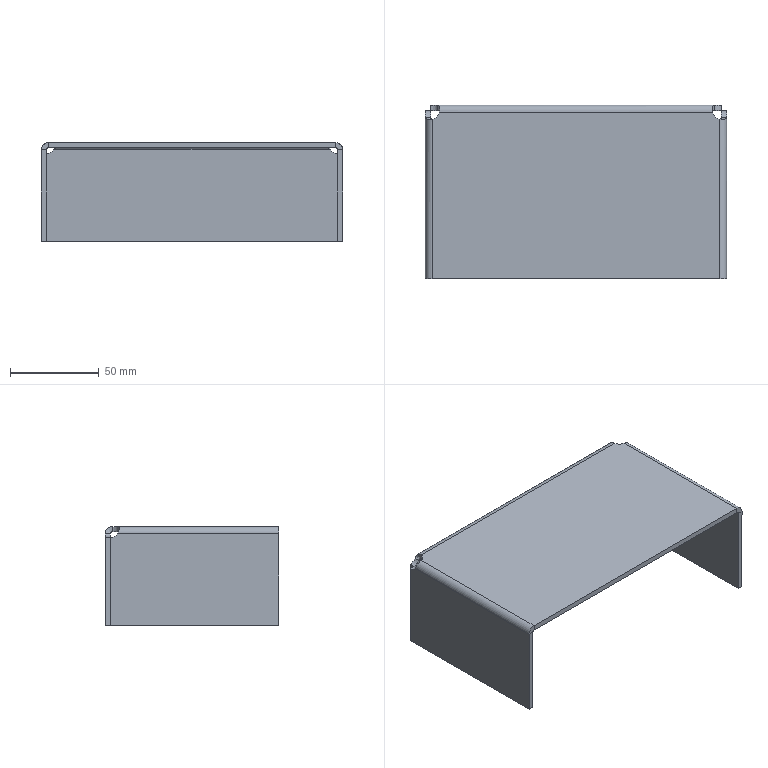Component | SolidWorks | ManualPumpProtectionBox-1 | 1 solid | 36 faces | volume 104585 mm3 | plane 20 | cylinder 12 | spline 4 | commonest cylinder face diameters 10 x6 2 x3 8 x3 | material Q235